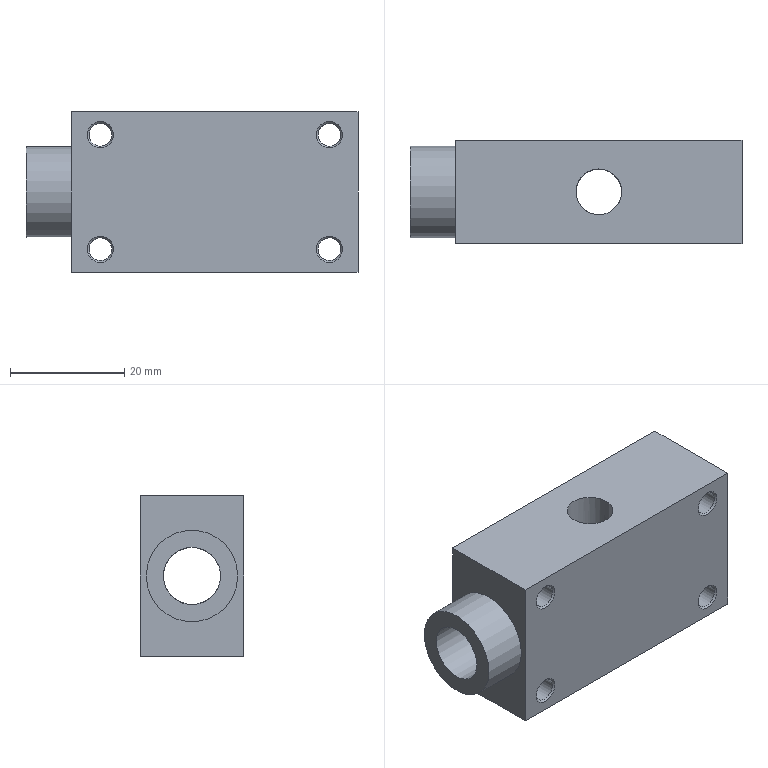Component | NX | SIDE_PISTON_CYLINDER | 1 solid | 21 faces | volume 20233 mm3 | cylinder 10 | plane 7 | cone 4 | commonest cylinder face diameters 4 x4 8 x2 5 x2 10 x1 16 x1